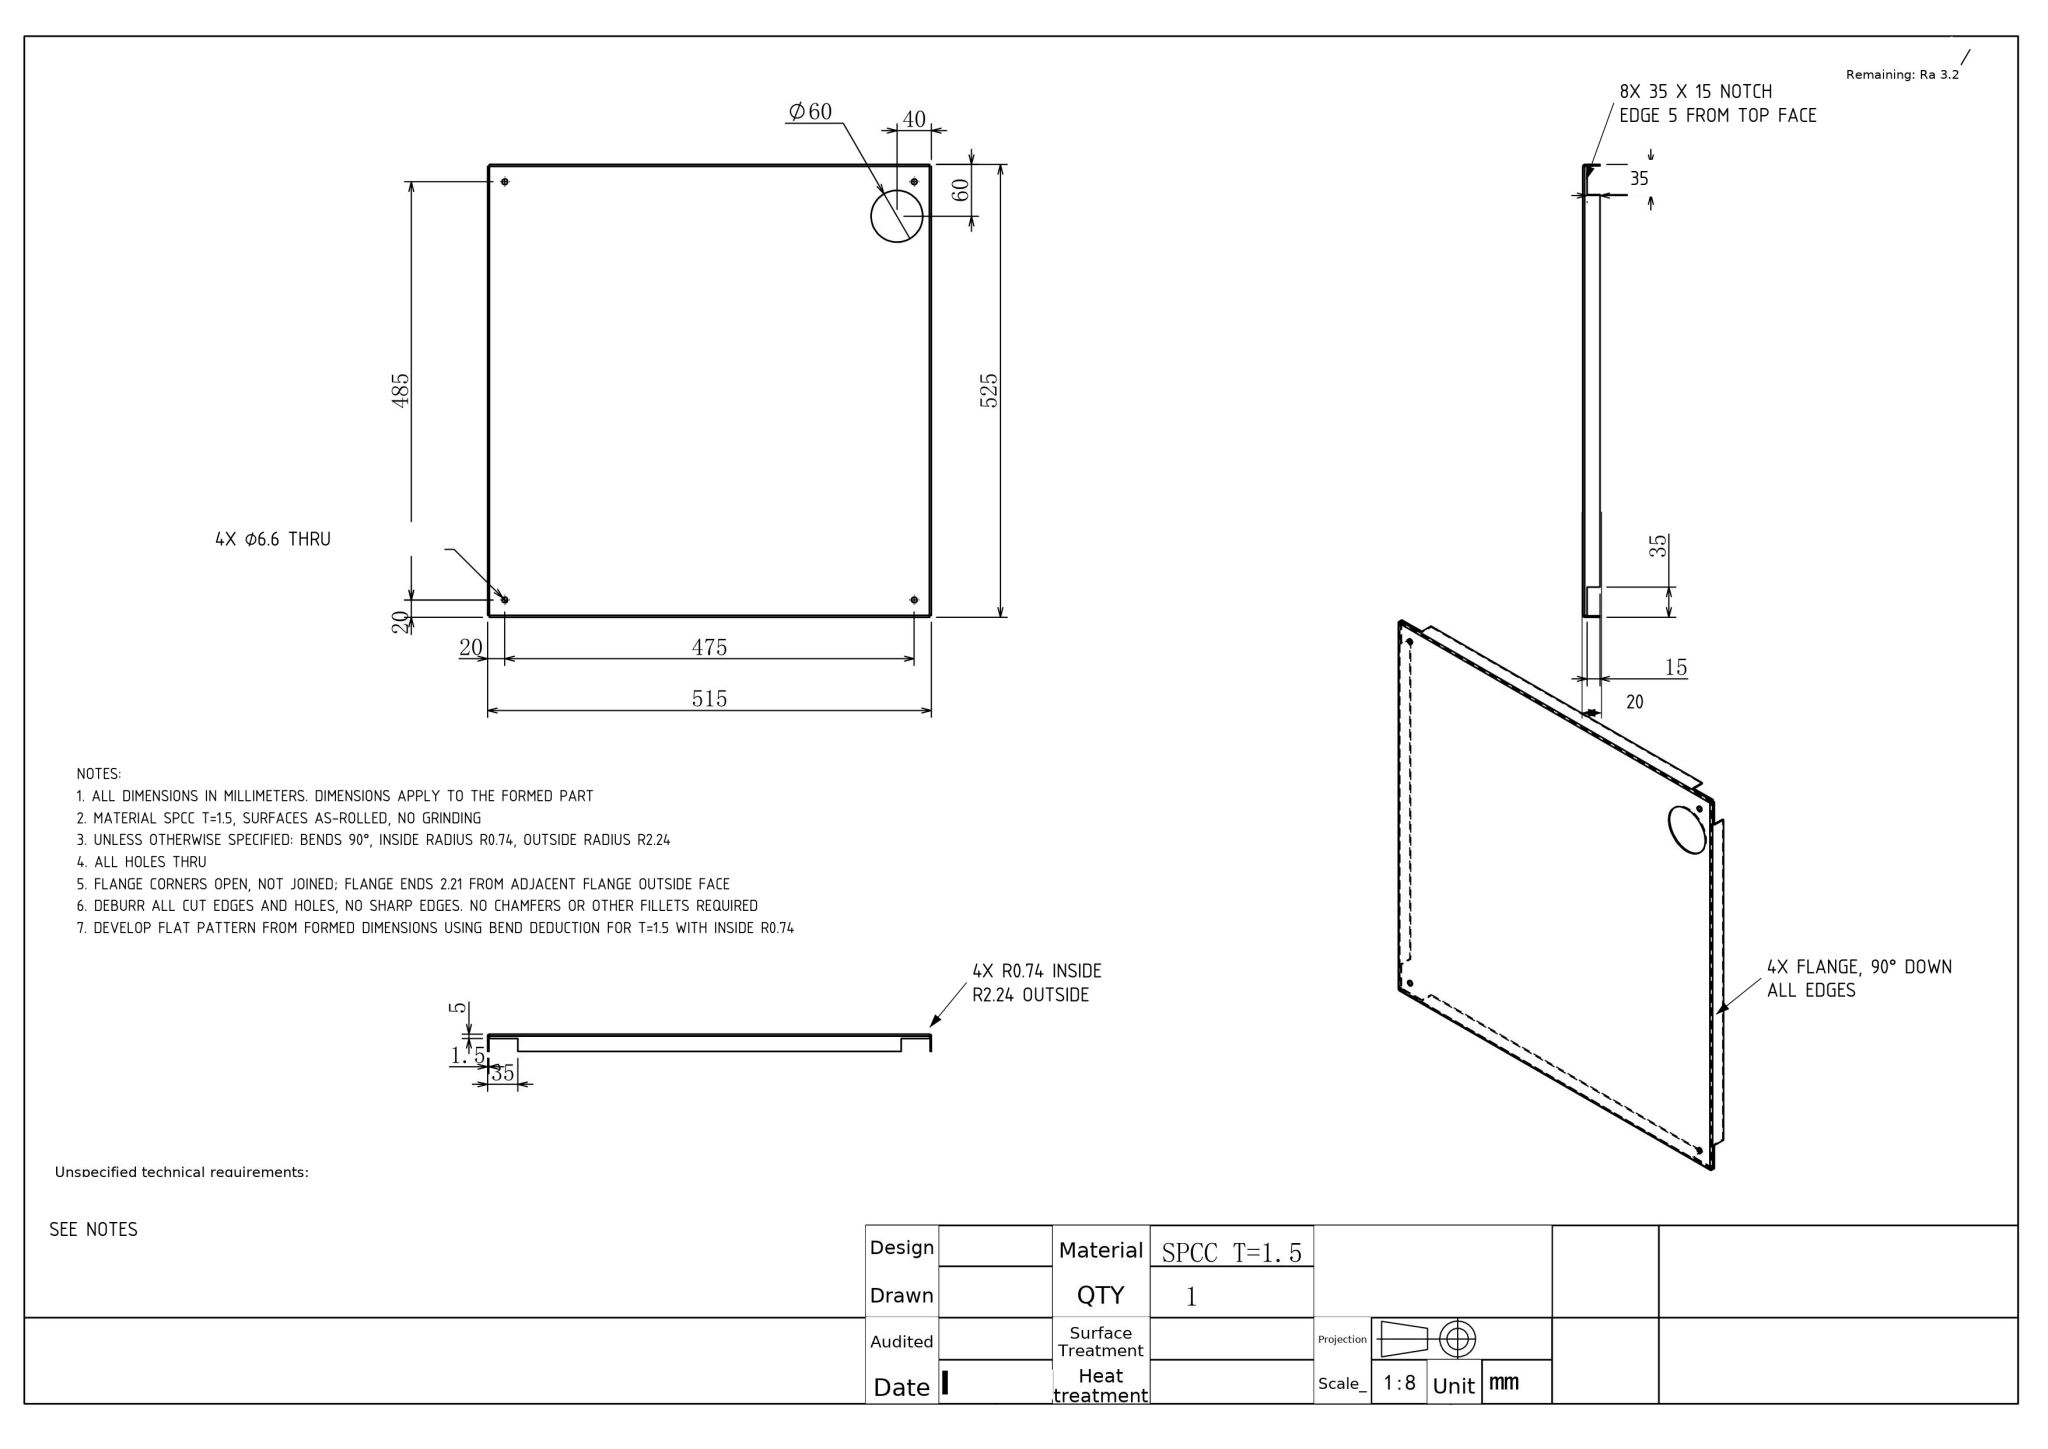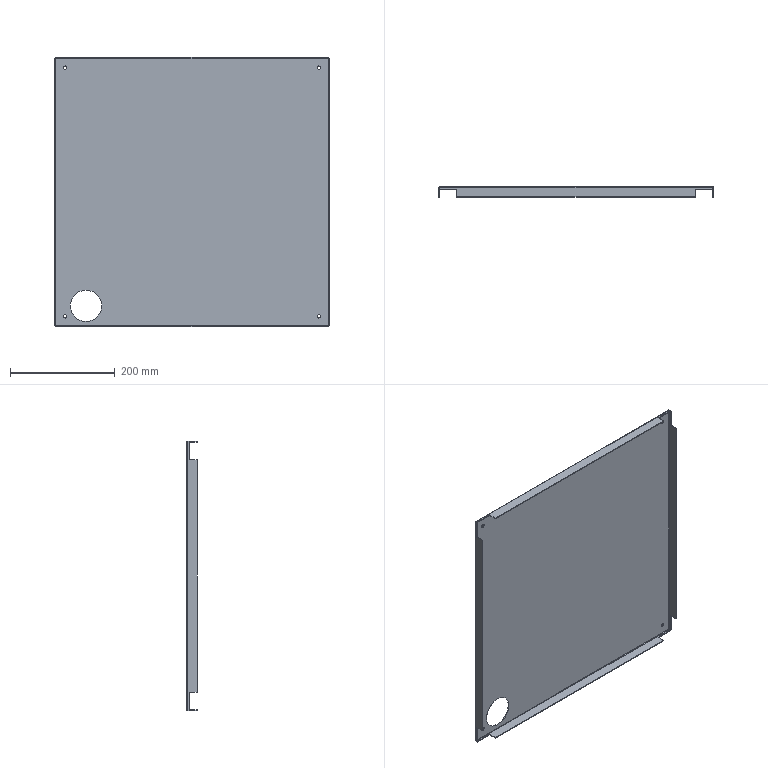Part | NX | mm | 1 solid | 64 faces | box 525 x 20 x 515 mm | volume 450440 mm3 | plane 38 | cylinder 18 | spline 8 | commonest cylinder face diameters 6.6 x8 4.473 x4 1.473 x4 60 x2